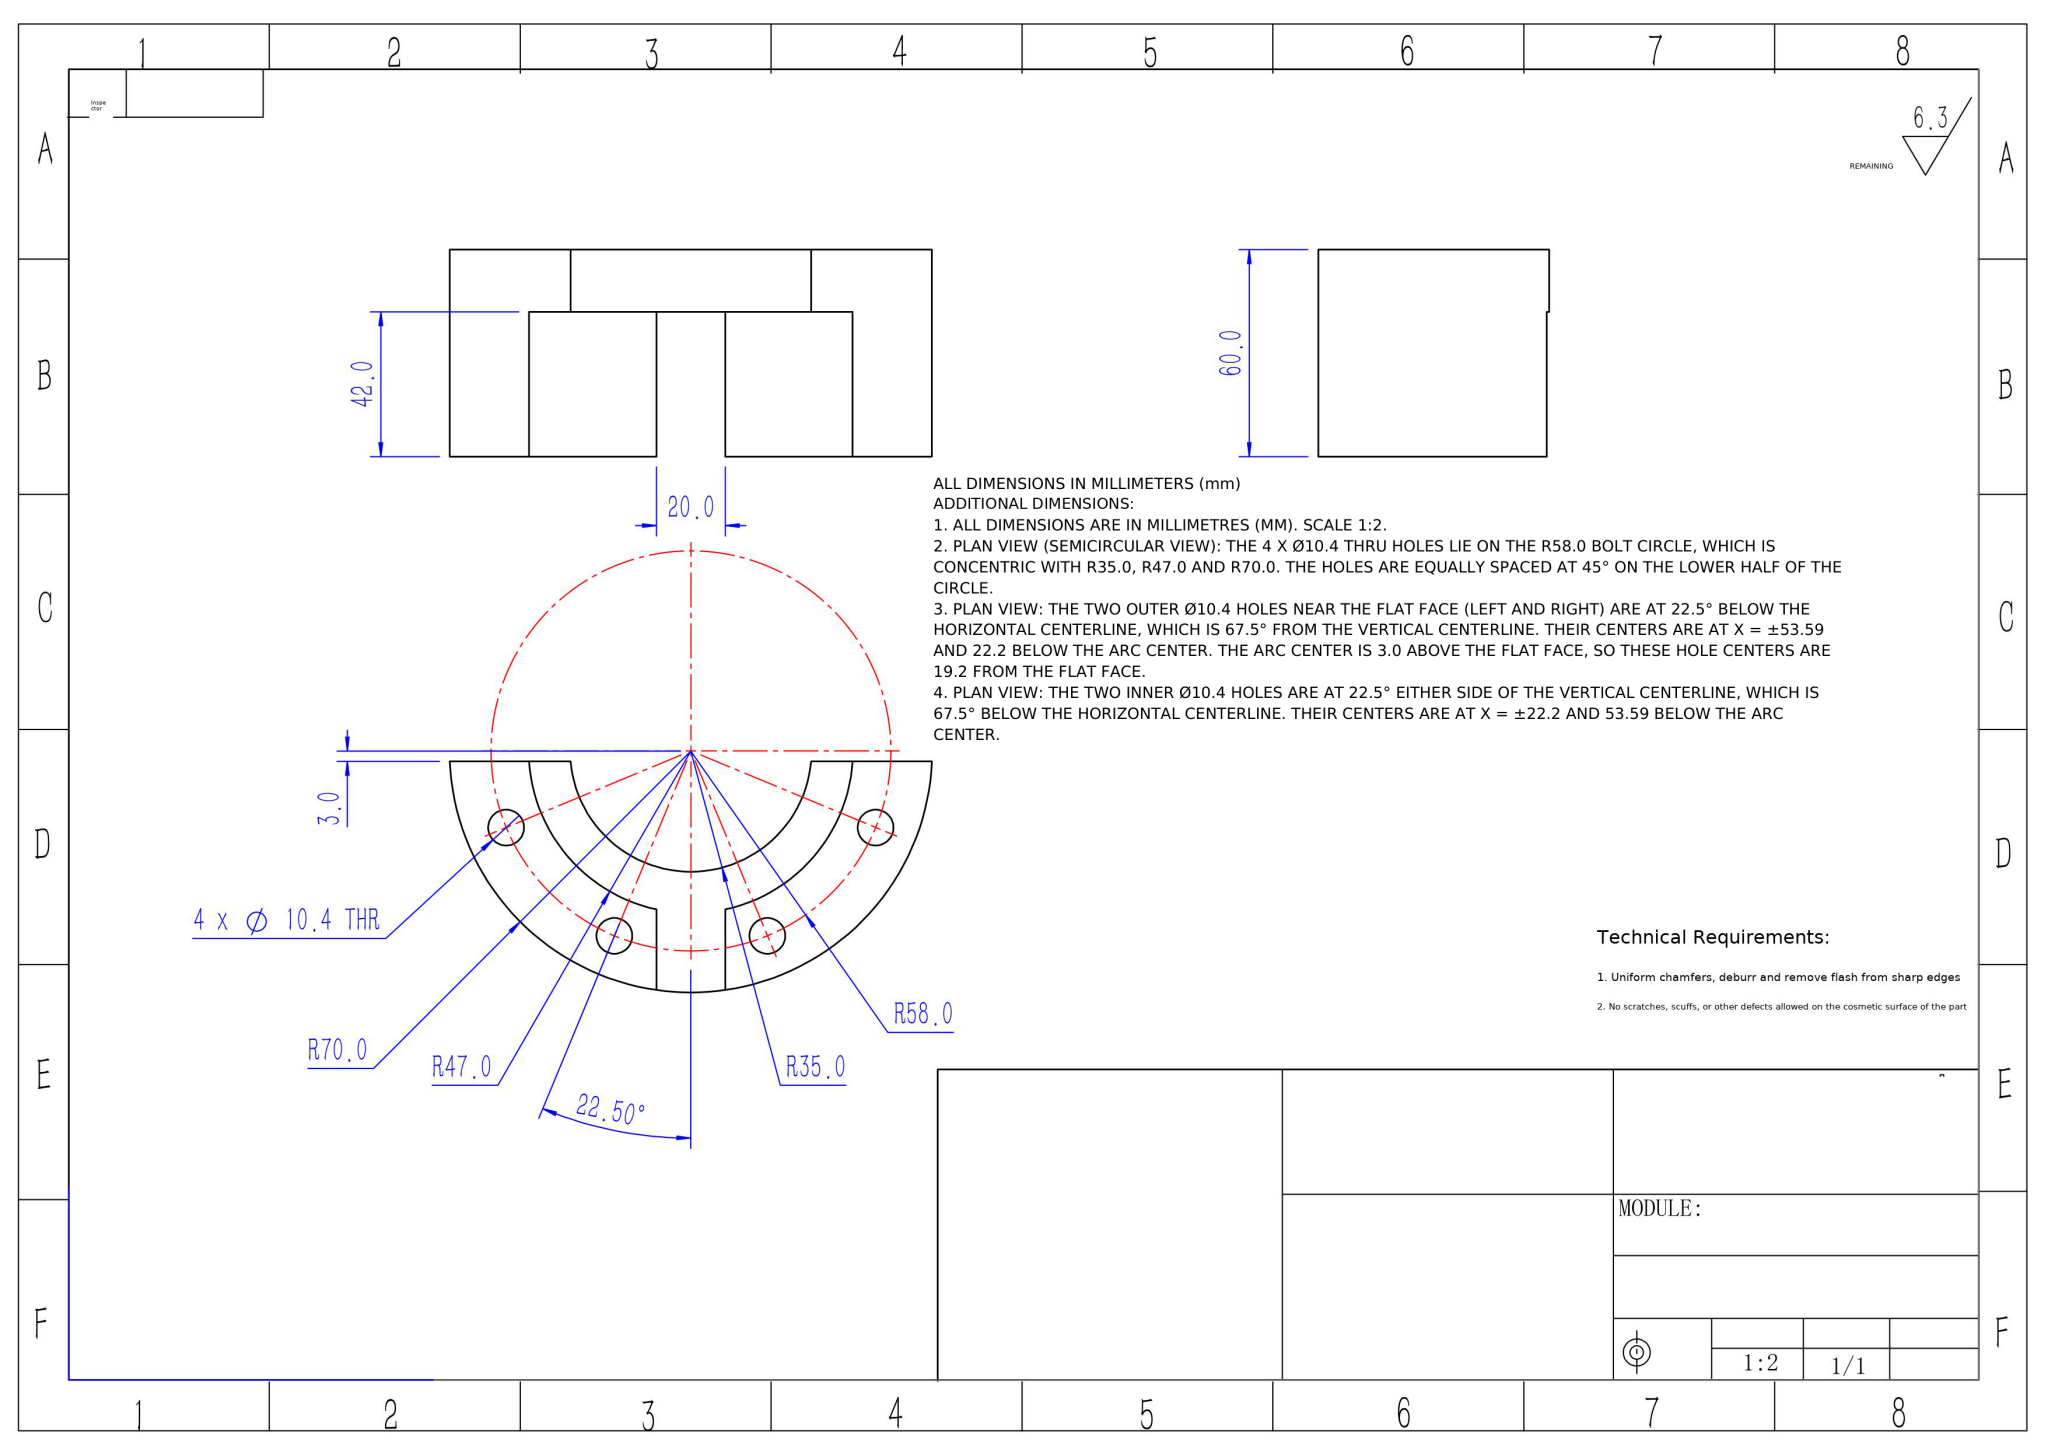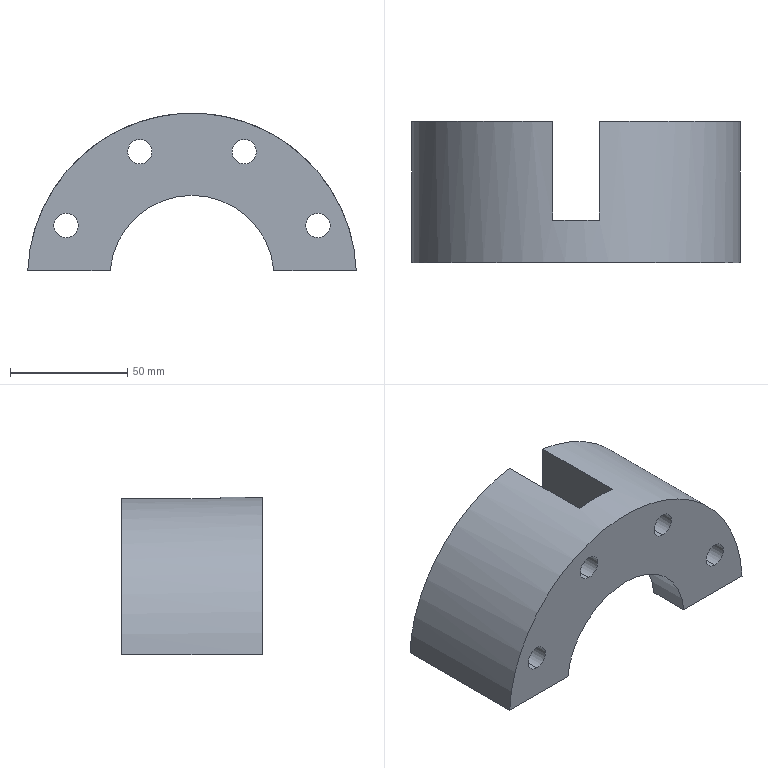Part | NX | mm | Curved Saddle Fork Bracket | 1 solid | 21 faces | box 139.87 x 60 x 67 mm | volume 232055 mm3 | cylinder 13 | plane 8 | commonest cylinder face diameters 10.4 x8 70 x2 94 x2 140 x1
STEP:
#1=CARTESIAN_POINT('',(53.585,60.,27.396));
#2=VERTEX_POINT('',#1);
#3=CARTESIAN_POINT('',(53.585,60.,16.996));
#4=VERTEX_POINT('',#3);
#5=CARTESIAN_POINT('',(53.585,60.,22.196));
#6=DIRECTION('',(-0.,-1.,0.));
#7=DIRECTION('',(0.,0.,-1.));
#8=AXIS2_PLACEMENT_3D('',#5,#6,#7);
#9=CIRCLE('',#8,5.2);
#10=EDGE_CURVE('',#2,#4,#9,.T.);
#11=ORIENTED_EDGE('',*,*,#10,.F.);
#12=CARTESIAN_POINT('',(53.585,0.,27.396));
#13=VERTEX_POINT('',#12);
#14=CARTESIAN_POINT('',(53.585,-0.,27.396));
#15=DIRECTION('',(-0.,-1.,0.));
#16=VECTOR('',#15,1000.);
#17=LINE('',#14,#16);
#18=EDGE_CURVE('',#2,#13,#17,.T.);
#19=ORIENTED_EDGE('',*,*,#18,.T.);
#20=CARTESIAN_POINT('',(53.585,0.,16.996));
#21=VERTEX_POINT('',#20);
#22=CARTESIAN_POINT('',(53.585,0.,22.196));
#23=DIRECTION('',(-0.,-1.,0.));
#24=DIRECTION('',(0.,0.,-1.));
#25=AXIS2_PLACEMENT_3D('',#22,#23,#24);
#26=CIRCLE('',#25,5.2);
#27=EDGE_CURVE('',#13,#21,#26,.T.);
#28=ORIENTED_EDGE('',*,*,#27,.T.);
#29=CARTESIAN_POINT('',(53.585,0.,16.996));
#30=DIRECTION('',(-0.,-1.,0.));
#31=VECTOR('',#30,1000.);
#32=LINE('',#29,#31);
#33=EDGE_CURVE('',#4,#21,#32,.T.);
#34=ORIENTED_EDGE('',*,*,#33,.F.);
#35=EDGE_LOOP('',(#11,#19,#28,#34));
#36=FACE_OUTER_BOUND('',#35,.T.);
#37=CARTESIAN_POINT('',(53.585,0.,22.196));
#38=DIRECTION('',(-0.,-1.,0.));
#39=DIRECTION('',(0.,0.,-1.));
#40=AXIS2_PLACEMENT_3D('',#37,#38,#39);
#41=CYLINDRICAL_SURFACE('',#40,5.2);
#42=ADVANCED_FACE('',(#36),#41,.F.);
#43=CARTESIAN_POINT('',(22.196,60.,58.785));
#44=VERTEX_POINT('',#43);
#45=CARTESIAN_POINT('',(22.196,60.,48.385));
#46=VERTEX_POINT('',#45);
#47=CARTESIAN_POINT('',(22.196,60.,53.585));
#48=DIRECTION('',(-0.,-1.,0.));
#49=DIRECTION('',(0.,0.,-1.));
#50=AXIS2_PLACEMENT_3D('',#47,#48,#49);
#51=CIRCLE('',#50,5.2);
#52=EDGE_CURVE('',#44,#46,#51,.T.);
#53=ORIENTED_EDGE('',*,*,#52,.F.);
#54=CARTESIAN_POINT('',(22.196,0.,58.785));
#55=VERTEX_POINT('',#54);
#56=CARTESIAN_POINT('',(22.196,-0.,58.785));
#57=DIRECTION('',(-0.,-1.,0.));
#58=VECTOR('',#57,1000.);
#59=LINE('',#56,#58);
#60=EDGE_CURVE('',#44,#55,#59,.T.);
#61=ORIENTED_EDGE('',*,*,#60,.T.);
#62=CARTESIAN_POINT('',(22.196,0.,48.385));
#63=VERTEX_POINT('',#62);
#64=CARTESIAN_POINT('',(22.196,0.,53.585));
#65=DIRECTION('',(-0.,-1.,0.));
#66=DIRECTION('',(0.,0.,-1.));
#67=AXIS2_PLACEMENT_3D('',#64,#65,#66);
#68=CIRCLE('',#67,5.2);
#69=EDGE_CURVE('',#55,#63,#68,.T.);
#70=ORIENTED_EDGE('',*,*,#69,.T.);
#71=CARTESIAN_POINT('',(22.196,0.,48.385));
#72=DIRECTION('',(-0.,-1.,0.));
#73=VECTOR('',#72,1000.);
#74=LINE('',#71,#73);
#75=EDGE_CURVE('',#46,#63,#74,.T.);
#76=ORIENTED_EDGE('',*,*,#75,.F.);
#77=EDGE_LOOP('',(#53,#61,#70,#76));
#78=FACE_OUTER_BOUND('',#77,.T.);
#79=CARTESIAN_POINT('',(22.196,0.,53.585));
#80=DIRECTION('',(-0.,-1.,0.));
#81=DIRECTION('',(0.,0.,-1.));
#82=AXIS2_PLACEMENT_3D('',#79,#80,#81);
#83=CYLINDRICAL_SURFACE('',#82,5.2);
#84=ADVANCED_FACE('',(#78),#83,.F.);
#85=CARTESIAN_POINT('',(-22.196,60.,58.785));
#86=VERTEX_POINT('',#85);
#87=CARTESIAN_POINT('',(-22.196,60.,48.385));
#88=VERTEX_POINT('',#87);
#89=CARTESIAN_POINT('',(-22.196,60.,53.585));
#90=DIRECTION('',(-0.,-1.,0.));
#91=DIRECTION('',(0.,0.,-1.));
#92=AXIS2_PLACEMENT_3D('',#89,#90,#91);
#93=CIRCLE('',#92,5.2);
#94=EDGE_CURVE('',#86,#88,#93,.T.);
#95=ORIENTED_EDGE('',*,*,#94,.F.);
#96=CARTESIAN_POINT('',(-22.196,0.,58.785));
#97=VERTEX_POINT('',#96);
#98=CARTESIAN_POINT('',(-22.196,-0.,58.785));
#99=DIRECTION('',(-0.,-1.,0.));
#100=VECTOR('',#99,1000.);
#101=LINE('',#98,#100);
#102=EDGE_CURVE('',#86,#97,#101,.T.);
#103=ORIENTED_EDGE('',*,*,#102,.T.);
#104=CARTESIAN_POINT('',(-22.196,0.,48.385));
#105=VERTEX_POINT('',#104);
#106=CARTESIAN_POINT('',(-22.196,0.,53.585));
#107=DIRECTION('',(-0.,-1.,0.));
#108=DIRECTION('',(0.,0.,-1.));
#109=AXIS2_PLACEMENT_3D('',#106,#107,#108);
#110=CIRCLE('',#109,5.2);
#111=EDGE_CURVE('',#97,#105,#110,.T.);
#112=ORIENTED_EDGE('',*,*,#111,.T.);
#113=CARTESIAN_POINT('',(-22.196,0.,48.385));
#114=DIRECTION('',(-0.,-1.,0.));
#115=VECTOR('',#114,1000.);
#116=LINE('',#113,#115);
#117=EDGE_CURVE('',#88,#105,#116,.T.);
#118=ORIENTED_EDGE('',*,*,#117,.F.);
#119=EDGE_LOOP('',(#95,#103,#112,#118));
#120=FACE_OUTER_BOUND('',#119,.T.);
#121=CARTESIAN_POINT('',(-22.196,0.,53.585));
#122=DIRECTION('',(-0.,-1.,0.));
#123=DIRECTION('',(0.,0.,-1.));
#124=AXIS2_PLACEMENT_3D('',#121,#122,#123);
#125=CYLINDRICAL_SURFACE('',#124,5.2);
#126=ADVANCED_FACE('',(#120),#125,.F.);
#127=CARTESIAN_POINT('',(-53.585,60.,27.396));
#128=VERTEX_POINT('',#127);
#129=CARTESIAN_POINT('',(-53.585,60.,16.996));
#130=VERTEX_POINT('',#129);
#131=CARTESIAN_POINT('',(-53.585,60.,22.196));
#132=DIRECTION('',(-0.,-1.,0.));
#133=DIRECTION('',(0.,0.,-1.));
#134=AXIS2_PLACEMENT_3D('',#131,#132,#133);
#135=CIRCLE('',#134,5.2);
#136=EDGE_CURVE('',#128,#130,#135,.T.);
#137=ORIENTED_EDGE('',*,*,#136,.F.);
#138=CARTESIAN_POINT('',(-53.585,0.,27.396));
#139=VERTEX_POINT('',#138);
#140=CARTESIAN_POINT('',(-53.585,-0.,27.396));
#141=DIRECTION('',(-0.,-1.,0.));
#142=VECTOR('',#141,1000.);
#143=LINE('',#140,#142);
#144=EDGE_CURVE('',#128,#139,#143,.T.);
#145=ORIENTED_EDGE('',*,*,#144,.T.);
#146=CARTESIAN_POINT('',(-53.585,0.,16.996));
#147=VERTEX_POINT('',#146);
#148=CARTESIAN_POINT('',(-53.585,0.,22.196));
#149=DIRECTION('',(-0.,-1.,0.));
#150=DIRECTION('',(0.,0.,-1.));
#151=AXIS2_PLACEMENT_3D('',#148,#149,#150);
#152=CIRCLE('',#151,5.2);
#153=EDGE_CURVE('',#139,#147,#152,.T.);
#154=ORIENTED_EDGE('',*,*,#153,.T.);
#155=CARTESIAN_POINT('',(-53.585,0.,16.996));
#156=DIRECTION('',(-0.,-1.,0.));
#157=VECTOR('',#156,1000.);
#158=LINE('',#155,#157);
#159=EDGE_CURVE('',#130,#147,#158,.T.);
#160=ORIENTED_EDGE('',*,*,#159,.F.);
#161=EDGE_LOOP('',(#137,#145,#154,#160));
#162=FACE_OUTER_BOUND('',#161,.T.);
#163=CARTESIAN_POINT('',(-53.585,0.,22.196));
#164=DIRECTION('',(-0.,-1.,0.));
#165=DIRECTION('',(0.,0.,-1.));
#166=AXIS2_PLACEMENT_3D('',#163,#164,#165);
#167=CYLINDRICAL_SURFACE('',#166,5.2);
#168=ADVANCED_FACE('',(#162),#167,.F.);
#169=CARTESIAN_POINT('',(-0.,0.,35.));
#170=VERTEX_POINT('',#169);
#171=CARTESIAN_POINT('',(34.871,0.,3.));
#172=VERTEX_POINT('',#171);
#173=CARTESIAN_POINT('',(0.,0.,0.));
#174=DIRECTION('',(0.,1.,-0.));
#175=DIRECTION('',(-0.,-0.,1.));
#176=AXIS2_PLACEMENT_3D('',#173,#174,#175);
#177=CIRCLE('',#176,35.);
#178=EDGE_CURVE('',#170,#172,#177,.T.);
#179=ORIENTED_EDGE('',*,*,#178,.F.);
#180=CARTESIAN_POINT('',(-0.,18.,35.));
#181=VERTEX_POINT('',#180);
#182=CARTESIAN_POINT('',(-0.,-0.,35.));
#183=DIRECTION('',(0.,1.,-0.));
#184=VECTOR('',#183,1000.);
#185=LINE('',#182,#184);
#186=EDGE_CURVE('',#170,#181,#185,.T.);
#187=ORIENTED_EDGE('',*,*,#186,.T.);
#188=CARTESIAN_POINT('',(34.871,18.,3.));
#189=VERTEX_POINT('',#188);
#190=CARTESIAN_POINT('',(0.,18.,0.));
#191=DIRECTION('',(0.,1.,-0.));
#192=DIRECTION('',(-0.,-0.,1.));
#193=AXIS2_PLACEMENT_3D('',#190,#191,#192);
#194=CIRCLE('',#193,35.);
#195=EDGE_CURVE('',#181,#189,#194,.T.);
#196=ORIENTED_EDGE('',*,*,#195,.T.);
#197=CARTESIAN_POINT('',(34.871,0.,3.));
#198=DIRECTION('',(-0.,-1.,0.));
#199=VECTOR('',#198,1000.);
#200=LINE('',#197,#199);
#201=EDGE_CURVE('',#189,#172,#200,.T.);
#202=ORIENTED_EDGE('',*,*,#201,.T.);
#203=EDGE_LOOP('',(#179,#187,#196,#202));
#204=FACE_OUTER_BOUND('',#203,.T.);
#205=CARTESIAN_POINT('',(0.,0.,0.));
#206=DIRECTION('',(0.,1.,-0.));
#207=DIRECTION('',(-0.,-0.,1.));
#208=AXIS2_PLACEMENT_3D('',#205,#206,#207);
#209=CYLINDRICAL_SURFACE('',#208,35.);
#210=ADVANCED_FACE('',(#204),#209,.F.);
#211=CARTESIAN_POINT('',(-10.,60.,69.282));
#212=VERTEX_POINT('',#211);
#213=CARTESIAN_POINT('',(-10.,60.,45.924));
#214=VERTEX_POINT('',#213);
#215=CARTESIAN_POINT('',(-10.,60.,70.));
#216=DIRECTION('',(0.,0.,-1.));
#217=VECTOR('',#216,1000.);
#218=LINE('',#215,#217);
#219=EDGE_CURVE('',#212,#214,#218,.T.);
#220=ORIENTED_EDGE('',*,*,#219,.T.);
#221=CARTESIAN_POINT('',(-46.904,60.,3.));
#222=VERTEX_POINT('',#221);
#223=CARTESIAN_POINT('',(0.,60.,0.));
#224=DIRECTION('',(0.,1.,-0.));
#225=DIRECTION('',(-0.,-0.,1.));
#226=AXIS2_PLACEMENT_3D('',#223,#224,#225);
#227=CIRCLE('',#226,47.);
#228=EDGE_CURVE('',#222,#214,#227,.T.);
#229=ORIENTED_EDGE('',*,*,#228,.F.);
#230=CARTESIAN_POINT('',(-69.936,60.,3.));
#231=VERTEX_POINT('',#230);
#232=CARTESIAN_POINT('',(-80.,60.,3.));
#233=DIRECTION('',(-1.,-0.,0.));
#234=VECTOR('',#233,1000.);
#235=LINE('',#232,#234);
#236=EDGE_CURVE('',#222,#231,#235,.T.);
#237=ORIENTED_EDGE('',*,*,#236,.T.);
#238=CARTESIAN_POINT('',(0.,60.,0.));
#239=DIRECTION('',(0.,1.,-0.));
#240=DIRECTION('',(-0.,-0.,1.));
#241=AXIS2_PLACEMENT_3D('',#238,#239,#240);
#242=CIRCLE('',#241,70.);
#243=EDGE_CURVE('',#231,#212,#242,.T.);
#244=ORIENTED_EDGE('',*,*,#243,.T.);
#245=EDGE_LOOP('',(#220,#229,#237,#244));
#246=FACE_OUTER_BOUND('',#245,.T.);
#247=CARTESIAN_POINT('',(-53.585,60.,22.196));
#248=DIRECTION('',(-0.,-1.,0.));
#249=DIRECTION('',(0.,0.,-1.));
#250=AXIS2_PLACEMENT_3D('',#247,#248,#249);
#251=CIRCLE('',#250,5.2);
#252=EDGE_CURVE('',#130,#128,#251,.T.);
#253=ORIENTED_EDGE('',*,*,#252,.T.);
#254=ORIENTED_EDGE('',*,*,#136,.T.);
#255=EDGE_LOOP('',(#253,#254));
#256=FACE_BOUND('',#255,.T.);
#257=CARTESIAN_POINT('',(-22.196,60.,53.585));
#258=DIRECTION('',(-0.,-1.,0.));
#259=DIRECTION('',(0.,0.,-1.));
#260=AXIS2_PLACEMENT_3D('',#257,#258,#259);
#261=CIRCLE('',#260,5.2);
#262=EDGE_CURVE('',#88,#86,#261,.T.);
#263=ORIENTED_EDGE('',*,*,#262,.T.);
#264=ORIENTED_EDGE('',*,*,#94,.T.);
#265=EDGE_LOOP('',(#263,#264));
#266=FACE_BOUND('',#265,.T.);
#267=CARTESIAN_POINT('',(0.,60.,0.));
#268=DIRECTION('',(0.,1.,0.));
#269=DIRECTION('',(-0.,-0.,1.));
#270=AXIS2_PLACEMENT_3D('',#267,#268,#269);
#271=PLANE('',#270);
#272=ADVANCED_FACE('',(#246,#256,#266),#271,.T.);
#273=ORIENTED_EDGE('',*,*,#228,.T.);
#274=CARTESIAN_POINT('',(-10.,18.,45.924));
#275=VERTEX_POINT('',#274);
#276=CARTESIAN_POINT('',(-10.,18.,45.924));
#277=DIRECTION('',(-0.,-1.,0.));
#278=VECTOR('',#277,1000.);
#279=LINE('',#276,#278);
#280=EDGE_CURVE('',#214,#275,#279,.T.);
#281=ORIENTED_EDGE('',*,*,#280,.T.);
#282=CARTESIAN_POINT('',(-46.904,18.,3.));
#283=VERTEX_POINT('',#282);
#284=CARTESIAN_POINT('',(0.,18.,0.));
#285=DIRECTION('',(0.,1.,-0.));
#286=DIRECTION('',(-0.,-0.,1.));
#287=AXIS2_PLACEMENT_3D('',#284,#285,#286);
#288=CIRCLE('',#287,47.);
#289=EDGE_CURVE('',#283,#275,#288,.T.);
#290=ORIENTED_EDGE('',*,*,#289,.F.);
#291=CARTESIAN_POINT('',(-46.904,18.,3.));
#292=DIRECTION('',(0.,1.,-0.));
#293=VECTOR('',#292,1000.);
#294=LINE('',#291,#293);
#295=EDGE_CURVE('',#283,#222,#294,.T.);
#296=ORIENTED_EDGE('',*,*,#295,.T.);
#297=EDGE_LOOP('',(#273,#281,#290,#296));
#298=FACE_OUTER_BOUND('',#297,.T.);
#299=CARTESIAN_POINT('',(0.,18.,0.));
#300=DIRECTION('',(0.,1.,-0.));
#301=DIRECTION('',(-0.,-0.,1.));
#302=AXIS2_PLACEMENT_3D('',#299,#300,#301);
#303=CYLINDRICAL_SURFACE('',#302,47.);
#304=ADVANCED_FACE('',(#298),#303,.F.);
#305=CARTESIAN_POINT('',(10.,60.,69.282));
#306=VERTEX_POINT('',#305);
#307=CARTESIAN_POINT('',(10.,18.,69.282));
#308=VERTEX_POINT('',#307);
#309=CARTESIAN_POINT('',(10.,60.,69.282));
#310=DIRECTION('',(-0.,-1.,0.));
#311=VECTOR('',#310,1000.);
#312=LINE('',#309,#311);
#313=EDGE_CURVE('',#306,#308,#312,.T.);
#314=ORIENTED_EDGE('',*,*,#313,.T.);
#315=CARTESIAN_POINT('',(-10.,18.,69.282));
#316=VERTEX_POINT('',#315);
#317=CARTESIAN_POINT('',(0.,18.,0.));
#318=DIRECTION('',(-0.,-1.,0.));
#319=DIRECTION('',(1.,-0.,-0.));
#320=AXIS2_PLACEMENT_3D('',#317,#318,#319);
#321=CIRCLE('',#320,70.);
#322=EDGE_CURVE('',#308,#316,#321,.T.);
#323=ORIENTED_EDGE('',*,*,#322,.T.);
#324=CARTESIAN_POINT('',(-10.,60.,69.282));
#325=DIRECTION('',(0.,1.,-0.));
#326=VECTOR('',#325,1000.);
#327=LINE('',#324,#326);
#328=EDGE_CURVE('',#316,#212,#327,.T.);
#329=ORIENTED_EDGE('',*,*,#328,.T.);
#330=ORIENTED_EDGE('',*,*,#243,.F.);
#331=CARTESIAN_POINT('',(-69.936,0.,3.));
#332=VERTEX_POINT('',#331);
#333=CARTESIAN_POINT('',(-69.936,60.,3.));
#334=DIRECTION('',(-0.,-1.,0.));
#335=VECTOR('',#334,1000.);
#336=LINE('',#333,#335);
#337=EDGE_CURVE('',#231,#332,#336,.T.);
#338=ORIENTED_EDGE('',*,*,#337,.T.);
#339=CARTESIAN_POINT('',(69.936,0.,3.));
#340=VERTEX_POINT('',#339);
#341=CARTESIAN_POINT('',(0.,0.,0.));
#342=DIRECTION('',(0.,1.,-0.));
#343=DIRECTION('',(-0.,-0.,1.));
#344=AXIS2_PLACEMENT_3D('',#341,#342,#343);
#345=CIRCLE('',#344,70.);
#346=EDGE_CURVE('',#332,#340,#345,.T.);
#347=ORIENTED_EDGE('',*,*,#346,.T.);
#348=CARTESIAN_POINT('',(69.936,60.,3.));
#349=VERTEX_POINT('',#348);
#350=CARTESIAN_POINT('',(69.936,60.,3.));
#351=DIRECTION('',(0.,1.,-0.));
#352=VECTOR('',#351,1000.);
#353=LINE('',#350,#352);
#354=EDGE_CURVE('',#340,#349,#353,.T.);
#355=ORIENTED_EDGE('',*,*,#354,.T.);
#356=CARTESIAN_POINT('',(0.,60.,0.));
#357=DIRECTION('',(0.,1.,-0.));
#358=DIRECTION('',(-0.,-0.,1.));
#359=AXIS2_PLACEMENT_3D('',#356,#357,#358);
#360=CIRCLE('',#359,70.);
#361=EDGE_CURVE('',#306,#349,#360,.T.);
#362=ORIENTED_EDGE('',*,*,#361,.F.);
#363=EDGE_LOOP('',(#314,#323,#329,#330,#338,#347,#355,#362));
#364=FACE_OUTER_BOUND('',#363,.T.);
#365=CARTESIAN_POINT('',(0.,60.,0.));
#366=DIRECTION('',(-0.,-1.,0.));
#367=DIRECTION('',(0.,0.,-1.));
#368=AXIS2_PLACEMENT_3D('',#365,#366,#367);
#369=CYLINDRICAL_SURFACE('',#368,70.);
#370=ADVANCED_FACE('',(#364),#369,.T.);
#371=CARTESIAN_POINT('',(10.,60.,45.924));
#372=VERTEX_POINT('',#371);
#373=CARTESIAN_POINT('',(10.,60.,70.));
#374=DIRECTION('',(0.,0.,-1.));
#375=VECTOR('',#374,1000.);
#376=LINE('',#373,#375);
#377=EDGE_CURVE('',#306,#372,#376,.T.);
#378=ORIENTED_EDGE('',*,*,#377,.F.);
#379=ORIENTED_EDGE('',*,*,#361,.T.);
#380=CARTESIAN_POINT('',(46.904,60.,3.));
#381=VERTEX_POINT('',#380);
#382=CARTESIAN_POINT('',(-80.,60.,3.));
#383=DIRECTION('',(-1.,-0.,0.));
#384=VECTOR('',#383,1000.);
#385=LINE('',#382,#384);
#386=EDGE_CURVE('',#349,#381,#385,.T.);
#387=ORIENTED_EDGE('',*,*,#386,.T.);
#388=CARTESIAN_POINT('',(0.,60.,0.));
#389=DIRECTION('',(0.,1.,-0.));
#390=DIRECTION('',(-0.,-0.,1.));
#391=AXIS2_PLACEMENT_3D('',#388,#389,#390);
#392=CIRCLE('',#391,47.);
#393=EDGE_CURVE('',#372,#381,#392,.T.);
#394=ORIENTED_EDGE('',*,*,#393,.F.);
#395=EDGE_LOOP('',(#378,#379,#387,#394));
#396=FACE_OUTER_BOUND('',#395,.T.);
#397=CARTESIAN_POINT('',(53.585,60.,22.196));
#398=DIRECTION('',(-0.,-1.,0.));
#399=DIRECTION('',(0.,0.,-1.));
#400=AXIS2_PLACEMENT_3D('',#397,#398,#399);
#401=CIRCLE('',#400,5.2);
#402=EDGE_CURVE('',#4,#2,#401,.T.);
#403=ORIENTED_EDGE('',*,*,#402,.T.);
#404=ORIENTED_EDGE('',*,*,#10,.T.);
#405=EDGE_LOOP('',(#403,#404));
#406=FACE_BOUND('',#405,.T.);
#407=CARTESIAN_POINT('',(22.196,60.,53.585));
#408=DIRECTION('',(-0.,-1.,0.));
#409=DIRECTION('',(0.,0.,-1.));
#410=AXIS2_PLACEMENT_3D('',#407,#408,#409);
#411=CIRCLE('',#410,5.2);
#412=EDGE_CURVE('',#46,#44,#411,.T.);
#413=ORIENTED_EDGE('',*,*,#412,.T.);
#414=ORIENTED_EDGE('',*,*,#52,.T.);
#415=EDGE_LOOP('',(#413,#414));
#416=FACE_BOUND('',#415,.T.);
#417=CARTESIAN_POINT('',(0.,60.,0.));
#418=DIRECTION('',(0.,1.,0.));
#419=DIRECTION('',(-0.,-0.,1.));
#420=AXIS2_PLACEMENT_3D('',#417,#418,#419);
#421=PLANE('',#420);
#422=ADVANCED_FACE('',(#396,#406,#416),#421,.T.);
#423=CARTESIAN_POINT('',(53.585,0.,22.196));
#424=DIRECTION('',(-0.,-1.,0.));
#425=DIRECTION('',(0.,0.,-1.));
#426=AXIS2_PLACEMENT_3D('',#423,#424,#425);
#427=CIRCLE('',#426,5.2);
#428=EDGE_CURVE('',#21,#13,#427,.T.);
#429=ORIENTED_EDGE('',*,*,#428,.F.);
#430=ORIENTED_EDGE('',*,*,#27,.F.);
#431=EDGE_LOOP('',(#429,#430));
#432=FACE_BOUND('',#431,.T.);
#433=CARTESIAN_POINT('',(22.196,0.,53.585));
#434=DIRECTION('',(-0.,-1.,0.));
#435=DIRECTION('',(0.,0.,-1.));
#436=AXIS2_PLACEMENT_3D('',#433,#434,#435);
#437=CIRCLE('',#436,5.2);
#438=EDGE_CURVE('',#63,#55,#437,.T.);
#439=ORIENTED_EDGE('',*,*,#438,.F.);
#440=ORIENTED_EDGE('',*,*,#69,.F.);
#441=EDGE_LOOP('',(#439,#440));
#442=FACE_BOUND('',#441,.T.);
#443=CARTESIAN_POINT('',(-22.196,0.,53.585));
#444=DIRECTION('',(-0.,-1.,0.));
#445=DIRECTION('',(0.,0.,-1.));
#446=AXIS2_PLACEMENT_3D('',#443,#444,#445);
#447=CIRCLE('',#446,5.2);
#448=EDGE_CURVE('',#105,#97,#447,.T.);
#449=ORIENTED_EDGE('',*,*,#448,.F.);
#450=ORIENTED_EDGE('',*,*,#111,.F.);
#451=EDGE_LOOP('',(#449,#450));
#452=FACE_BOUND('',#451,.T.);
#453=CARTESIAN_POINT('',(-53.585,0.,22.196));
#454=DIRECTION('',(-0.,-1.,0.));
#455=DIRECTION('',(0.,0.,-1.));
#456=AXIS2_PLACEMENT_3D('',#453,#454,#455);
#457=CIRCLE('',#456,5.2);
#458=EDGE_CURVE('',#147,#139,#457,.T.);
#459=ORIENTED_EDGE('',*,*,#458,.F.);
#460=ORIENTED_EDGE('',*,*,#153,.F.);
#461=EDGE_LOOP('',(#459,#460));
#462=FACE_BOUND('',#461,.T.);
#463=ORIENTED_EDGE('',*,*,#346,.F.);
#464=CARTESIAN_POINT('',(-34.871,0.,3.));
#465=VERTEX_POINT('',#464);
#466=CARTESIAN_POINT('',(-80.,0.,3.));
#467=DIRECTION('',(-1.,-0.,0.));
#468=VECTOR('',#467,1000.);
#469=LINE('',#466,#468);
#470=EDGE_CURVE('',#465,#332,#469,.T.);
#471=ORIENTED_EDGE('',*,*,#470,.F.);
#472=CARTESIAN_POINT('',(0.,0.,0.));
#473=DIRECTION('',(0.,1.,-0.));
#474=DIRECTION('',(-0.,-0.,1.));
#475=AXIS2_PLACEMENT_3D('',#472,#473,#474);
#476=CIRCLE('',#475,35.);
#477=EDGE_CURVE('',#465,#170,#476,.T.);
#478=ORIENTED_EDGE('',*,*,#477,.T.);
#479=ORIENTED_EDGE('',*,*,#178,.T.);
#480=CARTESIAN_POINT('',(-80.,0.,3.));
#481=DIRECTION('',(-1.,-0.,0.));
#482=VECTOR('',#481,1000.);
#483=LINE('',#480,#482);
#484=EDGE_CURVE('',#340,#172,#483,.T.);
#485=ORIENTED_EDGE('',*,*,#484,.F.);
#486=EDGE_LOOP('',(#463,#471,#478,#479,#485));
#487=FACE_OUTER_BOUND('',#486,.T.);
#488=CARTESIAN_POINT('',(0.,0.,0.));
#489=DIRECTION('',(0.,1.,0.));
#490=DIRECTION('',(-0.,-0.,1.));
#491=AXIS2_PLACEMENT_3D('',#488,#489,#490);
#492=PLANE('',#491);
#493=ADVANCED_FACE('',(#432,#442,#452,#462,#487),#492,.F.);
#494=CARTESIAN_POINT('',(10.,18.,45.924));
#495=VERTEX_POINT('',#494);
#496=CARTESIAN_POINT('',(46.904,18.,3.));
#497=VERTEX_POINT('',#496);
#498=CARTESIAN_POINT('',(0.,18.,0.));
#499=DIRECTION('',(0.,1.,-0.));
#500=DIRECTION('',(-0.,-0.,1.));
#501=AXIS2_PLACEMENT_3D('',#498,#499,#500);
#502=CIRCLE('',#501,47.);
#503=EDGE_CURVE('',#495,#497,#502,.T.);
#504=ORIENTED_EDGE('',*,*,#503,.F.);
#505=CARTESIAN_POINT('',(10.,18.,45.924));
#506=DIRECTION('',(0.,1.,-0.));
#507=VECTOR('',#506,1000.);
#508=LINE('',#505,#507);
#509=EDGE_CURVE('',#495,#372,#508,.T.);
#510=ORIENTED_EDGE('',*,*,#509,.T.);
#511=ORIENTED_EDGE('',*,*,#393,.T.);
#512=CARTESIAN_POINT('',(46.904,18.,3.));
#513=DIRECTION('',(-0.,-1.,0.));
#514=VECTOR('',#513,1000.);
#515=LINE('',#512,#514);
#516=EDGE_CURVE('',#381,#497,#515,.T.);
#517=ORIENTED_EDGE('',*,*,#516,.T.);
#518=EDGE_LOOP('',(#504,#510,#511,#517));
#519=FACE_OUTER_BOUND('',#518,.T.);
#520=CARTESIAN_POINT('',(0.,18.,0.));
#521=DIRECTION('',(0.,1.,-0.));
#522=DIRECTION('',(-0.,-0.,1.));
#523=AXIS2_PLACEMENT_3D('',#520,#521,#522);
#524=CYLINDRICAL_SURFACE('',#523,47.);
#525=ADVANCED_FACE('',(#519),#524,.F.);
#526=CARTESIAN_POINT('',(0.,18.,3.));
#527=DIRECTION('',(1.,0.,-0.));
#528=VECTOR('',#527,1000.);
#529=LINE('',#526,#528);
#530=EDGE_CURVE('',#189,#497,#529,.T.);
#531=ORIENTED_EDGE('',*,*,#530,.F.);
#532=ORIENTED_EDGE('',*,*,#195,.F.);
#533=CARTESIAN_POINT('',(-34.871,18.,3.));
#534=VERTEX_POINT('',#533);
#535=CARTESIAN_POINT('',(0.,18.,0.));
#536=DIRECTION('',(0.,1.,-0.));
#537=DIRECTION('',(-0.,-0.,1.));
#538=AXIS2_PLACEMENT_3D('',#535,#536,#537);
#539=CIRCLE('',#538,35.);
#540=EDGE_CURVE('',#534,#181,#539,.T.);
#541=ORIENTED_EDGE('',*,*,#540,.F.);
#542=CARTESIAN_POINT('',(0.,18.,3.));
#543=DIRECTION('',(1.,0.,-0.));
#544=VECTOR('',#543,1000.);
#545=LINE('',#542,#544);
#546=EDGE_CURVE('',#283,#534,#545,.T.);
#547=ORIENTED_EDGE('',*,*,#546,.F.);
#548=ORIENTED_EDGE('',*,*,#289,.T.);
#549=CARTESIAN_POINT('',(-10.,18.,70.));
#550=DIRECTION('',(0.,0.,-1.));
#551=VECTOR('',#550,1000.);
#552=LINE('',#549,#551);
#553=EDGE_CURVE('',#316,#275,#552,.T.);
#554=ORIENTED_EDGE('',*,*,#553,.F.);
#555=ORIENTED_EDGE('',*,*,#322,.F.);
#556=CARTESIAN_POINT('',(10.,18.,70.));
#557=DIRECTION('',(0.,0.,-1.));
#558=VECTOR('',#557,1000.);
#559=LINE('',#556,#558);
#560=EDGE_CURVE('',#308,#495,#559,.T.);
#561=ORIENTED_EDGE('',*,*,#560,.T.);
#562=ORIENTED_EDGE('',*,*,#503,.T.);
#563=EDGE_LOOP('',(#531,#532,#541,#547,#548,#554,#555,#561,#562));
#564=FACE_OUTER_BOUND('',#563,.T.);
#565=CARTESIAN_POINT('',(0.,18.,0.));
#566=DIRECTION('',(0.,1.,0.));
#567=DIRECTION('',(-0.,-0.,1.));
#568=AXIS2_PLACEMENT_3D('',#565,#566,#567);
#569=PLANE('',#568);
#570=ADVANCED_FACE('',(#564),#569,.T.);
#571=ORIENTED_EDGE('',*,*,#186,.F.);
#572=ORIENTED_EDGE('',*,*,#477,.F.);
#573=CARTESIAN_POINT('',(-34.871,0.,3.));
#574=DIRECTION('',(0.,1.,-0.));
#575=VECTOR('',#574,1000.);
#576=LINE('',#573,#575);
#577=EDGE_CURVE('',#465,#534,#576,.T.);
#578=ORIENTED_EDGE('',*,*,#577,.T.);
#579=ORIENTED_EDGE('',*,*,#540,.T.);
#580=EDGE_LOOP('',(#571,#572,#578,#579));
#581=FACE_OUTER_BOUND('',#580,.T.);
#582=CARTESIAN_POINT('',(0.,0.,0.));
#583=DIRECTION('',(0.,1.,-0.));
#584=DIRECTION('',(-0.,-0.,1.));
#585=AXIS2_PLACEMENT_3D('',#582,#583,#584);
#586=CYLINDRICAL_SURFACE('',#585,35.);
#587=ADVANCED_FACE('',(#581),#586,.F.);
#588=ORIENTED_EDGE('',*,*,#236,.F.);
#589=ORIENTED_EDGE('',*,*,#295,.F.);
#590=ORIENTED_EDGE('',*,*,#546,.T.);
#591=ORIENTED_EDGE('',*,*,#577,.F.);
#592=ORIENTED_EDGE('',*,*,#470,.T.);
#593=ORIENTED_EDGE('',*,*,#337,.F.);
#594=EDGE_LOOP('',(#588,#589,#590,#591,#592,#593));
#595=FACE_OUTER_BOUND('',#594,.T.);
#596=CARTESIAN_POINT('',(-80.,60.,3.));
#597=DIRECTION('',(0.,-0.,1.));
#598=DIRECTION('',(1.,0.,-0.));
#599=AXIS2_PLACEMENT_3D('',#596,#597,#598);
#600=PLANE('',#599);
#601=ADVANCED_FACE('',(#595),#600,.F.);
#602=ORIENTED_EDGE('',*,*,#484,.T.);
#603=ORIENTED_EDGE('',*,*,#201,.F.);
#604=ORIENTED_EDGE('',*,*,#530,.T.);
#605=ORIENTED_EDGE('',*,*,#516,.F.);
#606=ORIENTED_EDGE('',*,*,#386,.F.);
#607=ORIENTED_EDGE('',*,*,#354,.F.);
#608=EDGE_LOOP('',(#602,#603,#604,#605,#606,#607));
#609=FACE_OUTER_BOUND('',#608,.T.);
#610=CARTESIAN_POINT('',(-80.,60.,3.));
#611=DIRECTION('',(0.,-0.,1.));
#612=DIRECTION('',(1.,0.,-0.));
#613=AXIS2_PLACEMENT_3D('',#610,#611,#612);
#614=PLANE('',#613);
#615=ADVANCED_FACE('',(#609),#614,.F.);
#616=ORIENTED_EDGE('',*,*,#144,.F.);
#617=ORIENTED_EDGE('',*,*,#252,.F.);
#618=ORIENTED_EDGE('',*,*,#159,.T.);
#619=ORIENTED_EDGE('',*,*,#458,.T.);
#620=EDGE_LOOP('',(#616,#617,#618,#619));
#621=FACE_OUTER_BOUND('',#620,.T.);
#622=CARTESIAN_POINT('',(-53.585,0.,22.196));
#623=DIRECTION('',(-0.,-1.,0.));
#624=DIRECTION('',(0.,0.,-1.));
#625=AXIS2_PLACEMENT_3D('',#622,#623,#624);
#626=CYLINDRICAL_SURFACE('',#625,5.2);
#627=ADVANCED_FACE('',(#621),#626,.F.);
#628=ORIENTED_EDGE('',*,*,#102,.F.);
#629=ORIENTED_EDGE('',*,*,#262,.F.);
#630=ORIENTED_EDGE('',*,*,#117,.T.);
#631=ORIENTED_EDGE('',*,*,#448,.T.);
#632=EDGE_LOOP('',(#628,#629,#630,#631));
#633=FACE_OUTER_BOUND('',#632,.T.);
#634=CARTESIAN_POINT('',(-22.196,0.,53.585));
#635=DIRECTION('',(-0.,-1.,0.));
#636=DIRECTION('',(0.,0.,-1.));
#637=AXIS2_PLACEMENT_3D('',#634,#635,#636);
#638=CYLINDRICAL_SURFACE('',#637,5.2);
#639=ADVANCED_FACE('',(#633),#638,.F.);
#640=ORIENTED_EDGE('',*,*,#60,.F.);
#641=ORIENTED_EDGE('',*,*,#412,.F.);
#642=ORIENTED_EDGE('',*,*,#75,.T.);
#643=ORIENTED_EDGE('',*,*,#438,.T.);
#644=EDGE_LOOP('',(#640,#641,#642,#643));
#645=FACE_OUTER_BOUND('',#644,.T.);
#646=CARTESIAN_POINT('',(22.196,0.,53.585));
#647=DIRECTION('',(-0.,-1.,0.));
#648=DIRECTION('',(0.,0.,-1.));
#649=AXIS2_PLACEMENT_3D('',#646,#647,#648);
#650=CYLINDRICAL_SURFACE('',#649,5.2);
#651=ADVANCED_FACE('',(#645),#650,.F.);
#652=ORIENTED_EDGE('',*,*,#18,.F.);
#653=ORIENTED_EDGE('',*,*,#402,.F.);
#654=ORIENTED_EDGE('',*,*,#33,.T.);
#655=ORIENTED_EDGE('',*,*,#428,.T.);
#656=EDGE_LOOP('',(#652,#653,#654,#655));
#657=FACE_OUTER_BOUND('',#656,.T.);
#658=CARTESIAN_POINT('',(53.585,0.,22.196));
#659=DIRECTION('',(-0.,-1.,0.));
#660=DIRECTION('',(0.,0.,-1.));
#661=AXIS2_PLACEMENT_3D('',#658,#659,#660);
#662=CYLINDRICAL_SURFACE('',#661,5.2);
#663=ADVANCED_FACE('',(#657),#662,.F.);
#664=ORIENTED_EDGE('',*,*,#553,.T.);
#665=ORIENTED_EDGE('',*,*,#280,.F.);
#666=ORIENTED_EDGE('',*,*,#219,.F.);
#667=ORIENTED_EDGE('',*,*,#328,.F.);
#668=EDGE_LOOP('',(#664,#665,#666,#667));
#669=FACE_OUTER_BOUND('',#668,.T.);
#670=CARTESIAN_POINT('',(-10.,18.,70.));
#671=DIRECTION('',(-1.,-0.,-0.));
#672=DIRECTION('',(-0.,-0.,1.));
#673=AXIS2_PLACEMENT_3D('',#670,#671,#672);
#674=PLANE('',#673);
#675=ADVANCED_FACE('',(#669),#674,.F.);
#676=ORIENTED_EDGE('',*,*,#377,.T.);
#677=ORIENTED_EDGE('',*,*,#509,.F.);
#678=ORIENTED_EDGE('',*,*,#560,.F.);
#679=ORIENTED_EDGE('',*,*,#313,.F.);
#680=EDGE_LOOP('',(#676,#677,#678,#679));
#681=FACE_OUTER_BOUND('',#680,.T.);
#682=CARTESIAN_POINT('',(10.,18.,70.));
#683=DIRECTION('',(1.,0.,0.));
#684=DIRECTION('',(0.,0.,-1.));
#685=AXIS2_PLACEMENT_3D('',#682,#683,#684);
#686=PLANE('',#685);
#687=ADVANCED_FACE('',(#681),#686,.F.);
#688=CLOSED_SHELL('',(#42,#84,#126,#168,#210,#272,#304,#370,#422,#493,#525,#570,#587,#601,#615,#627,#639,#651,#663,#675,#687));
#689=MANIFOLD_SOLID_BREP('',#688);
#690=CARTESIAN_POINT('',(0.,0.,0.));
#691=DIRECTION('',(0.,0.,1.));
#692=DIRECTION('',(1.,0.,0.));
#693=AXIS2_PLACEMENT_3D('',#690,#691,#692);
#694=(LENGTH_UNIT()NAMED_UNIT(*)SI_UNIT(.MILLI.,.METRE.));
#695=UNCERTAINTY_MEASURE_WITH_UNIT(LENGTH_MEASURE(0.00001),#694,'','');
#696=(NAMED_UNIT(*)PLANE_ANGLE_UNIT()SI_UNIT($,.RADIAN.));
#697=(NAMED_UNIT(*)SI_UNIT($,.STERADIAN.)SOLID_ANGLE_UNIT());
#698=(GEOMETRIC_REPRESENTATION_CONTEXT(3)GLOBAL_UNCERTAINTY_ASSIGNED_CONTEXT((#695))GLOBAL_UNIT_ASSIGNED_CONTEXT((#694,#696,#697))REPRESENTATION_CONTEXT('',''));
#699=ADVANCED_BREP_SHAPE_REPRESENTATION('',(#689,#693),#698);
#700=COLOUR_RGB('',0.7922,0.8196,0.9333);
#701=FILL_AREA_STYLE_COLOUR('',#700);
#702=FILL_AREA_STYLE('',(#701));
#703=SURFACE_STYLE_FILL_AREA(#702);
#704=SURFACE_SIDE_STYLE('',(#703));
#705=SURFACE_STYLE_USAGE(.BOTH.,#704);
#706=PRESENTATION_STYLE_ASSIGNMENT((#705));
#707=STYLED_ITEM('',(#706),#689);
#708=PRESENTATION_LAYER_ASSIGNMENT('','',(#707));
#709=(LENGTH_UNIT()NAMED_UNIT(*)SI_UNIT(.MILLI.,.METRE.));
#710=UNCERTAINTY_MEASURE_WITH_UNIT(LENGTH_MEASURE(0.00001),#709,'','');
#711=(NAMED_UNIT(*)PLANE_ANGLE_UNIT()SI_UNIT($,.RADIAN.));
#712=(NAMED_UNIT(*)SI_UNIT($,.STERADIAN.)SOLID_ANGLE_UNIT());
#713=(GEOMETRIC_REPRESENTATION_CONTEXT(3)GLOBAL_UNCERTAINTY_ASSIGNED_CONTEXT((#710))GLOBAL_UNIT_ASSIGNED_CONTEXT((#709,#711,#712))REPRESENTATION_CONTEXT('',''));
#714=MECHANICAL_DESIGN_GEOMETRIC_PRESENTATION_REPRESENTATION('',(#707),#713);